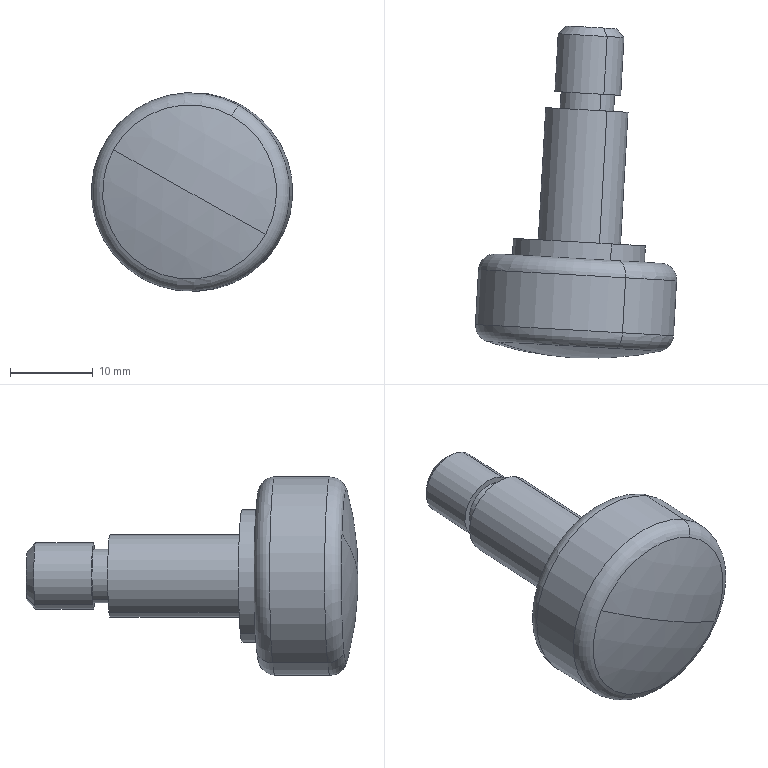Component | SolidWorks | Foot-1 | 1 solid | 23 faces | box 24.34 x 40.17 x 24 mm | volume 7037 mm3 | cylinder 10 | plane 5 | torus 4 | cone 2 | sphere 2 | commonest cylinder face diameters 24 x2 16 x2 10 x2 6.5 x2 8 x2
build123d program:
from build123d import *

# Parameters (mm, degrees)
CHAMFER1_SIZE = 1


with BuildPart() as part:
    # Sketch1 → Revolve1 (revolve)
    with BuildSketch(Plane.XY, mode=Mode.PRIVATE) as revolve1_sk:
        with BuildLine():
            Line((3.339, 12), (10, 12))
            ThreePointArc((10, 12), (11.414, 11.414), (12, 10))
            Line((12, 10), (12, 8))
            Line((12, 8), (14, 8))
            Line((14, 8), (14, 5))
            Line((14, 5), (30, 5))
            Line((30, 5), (30, 3.25))
            Line((30, 3.25), (32, 3.25))
            Line((32, 3.25), (32, 4))
            Line((32, 4), (40, 4))
            Line((40, 4), (40, 0))
            Line((40, 0), (0, 0))
            ThreePointArc((0, 0), (0.354, 5.31), (1.41, 10.526))
            ThreePointArc((1.41, 10.526), (2.125, 11.589), (3.339, 12))
        make_face()
    revolve(revolve1_sk.sketch.rotate(Axis((0, 0, 0), (1, 0, 0)), 90), axis=Axis((0, 0, 0), (1, 0, 0)))

    # Chamfer1
    chamfer1_edges = [part.edges().sort_by_distance(p)[0] for p in [
        (40, 0, -4),
    ]]
    chamfer(chamfer1_edges, length=CHAMFER1_SIZE)


solid = part.part

# Placed as in the assembly
solid = solid.moved(Location((194.855, -53.332, 1009), (-178.207, -28.965, -86.302)))
STEP:
#1=COLOUR_RGB('',0.7922,0.8196,0.9333);
#2=FILL_AREA_STYLE_COLOUR('',#1);
#3=FILL_AREA_STYLE('',(#2));
#4=SURFACE_STYLE_FILL_AREA(#3);
#5=SURFACE_SIDE_STYLE('',(#4));
#6=SURFACE_STYLE_USAGE(.BOTH.,#5);
#7=PRESENTATION_STYLE_ASSIGNMENT((#6));
#8=CARTESIAN_POINT('',(7.703,-0.5241,39.621));
#9=VERTEX_POINT('',#8);
#10=CARTESIAN_POINT('',(7.818,-0.5306,39.828));
#11=VERTEX_POINT('',#10);
#12=CARTESIAN_POINT('',(7.76,-0.5274,39.724));
#13=DIRECTION('',(0.05643,0.9984,0.));
#14=DIRECTION('',(0.4842,-0.02737,0.8745));
#15=AXIS2_PLACEMENT_3D('',#12,#13,#14);
#16=CIRCLE('',#15,0.1181);
#17=EDGE_CURVE('',#9,#11,#16,.T.);
#18=ORIENTED_EDGE('',*,*,#17,.F.);
#19=CARTESIAN_POINT('',(7.682,-0.5624,39.587));
#20=VERTEX_POINT('',#19);
#21=CARTESIAN_POINT('',(7.682,-0.5624,39.587));
#22=DIRECTION('',(-0.3823,-0.6866,-0.6184));
#23=VECTOR('',#22,39.37);
#24=LINE('',#21,#23);
#25=EDGE_CURVE('',#9,#20,#24,.T.);
#26=ORIENTED_EDGE('',*,*,#25,.T.);
#27=CARTESIAN_POINT('',(7.834,-0.571,39.862));
#28=VERTEX_POINT('',#27);
#29=CARTESIAN_POINT('',(7.758,-0.5667,39.724));
#30=DIRECTION('',(-0.05643,-0.9984,-0.));
#31=DIRECTION('',(0.4842,-0.02737,0.8745));
#32=AXIS2_PLACEMENT_3D('',#29,#30,#31);
#33=CIRCLE('',#32,0.1575);
#34=EDGE_CURVE('',#28,#20,#33,.T.);
#35=ORIENTED_EDGE('',*,*,#34,.F.);
#36=CARTESIAN_POINT('',(7.834,-0.571,39.862));
#37=DIRECTION('',(0.3025,-0.7253,0.6184));
#38=VECTOR('',#37,39.37);
#39=LINE('',#36,#38);
#40=EDGE_CURVE('',#11,#28,#39,.T.);
#41=ORIENTED_EDGE('',*,*,#40,.F.);
#42=EDGE_LOOP('',(#18,#26,#35,#41));
#43=FACE_OUTER_BOUND('',#42,.T.);
#44=CARTESIAN_POINT('',(7.758,-0.5667,39.724));
#45=DIRECTION('',(-0.05643,-0.9984,-0.));
#46=DIRECTION('',(0.4842,-0.02737,0.8745));
#47=AXIS2_PLACEMENT_3D('',#44,#45,#46);
#48=CONICAL_SURFACE('',#47,0.1575,0.7854);
#49=ADVANCED_FACE('',(#43),#48,.T.);
#50=CARTESIAN_POINT('',(7.908,-1.981,40.138));
#51=VERTEX_POINT('',#50);
#52=CARTESIAN_POINT('',(7.45,-1.955,39.311));
#53=VERTEX_POINT('',#52);
#54=CARTESIAN_POINT('',(7.679,-1.968,39.724));
#55=DIRECTION('',(-0.05643,-0.9984,-0.));
#56=DIRECTION('',(0.4842,-0.02737,0.8745));
#57=AXIS2_PLACEMENT_3D('',#54,#55,#56);
#58=CIRCLE('',#57,0.4724);
#59=EDGE_CURVE('',#51,#53,#58,.T.);
#60=ORIENTED_EDGE('',*,*,#59,.T.);
#61=CARTESIAN_POINT('',(7.474,-2.033,39.362));
#62=VERTEX_POINT('',#61);
#63=CARTESIAN_POINT('',(7.488,-1.958,39.38));
#64=DIRECTION('',(-0.8731,0.04935,0.485));
#65=DIRECTION('',(0.4856,0.,0.8742));
#66=AXIS2_PLACEMENT_3D('',#63,#64,#65);
#67=CIRCLE('',#66,0.07874);
#68=EDGE_CURVE('',#53,#62,#67,.T.);
#69=ORIENTED_EDGE('',*,*,#68,.T.);
#70=CARTESIAN_POINT('',(7.313,-2.024,39.925));
#71=VERTEX_POINT('',#70);
#72=CARTESIAN_POINT('',(7.675,-2.044,39.724));
#73=DIRECTION('',(-0.05643,-0.9984,-0.));
#74=DIRECTION('',(0.4842,-0.02737,0.8745));
#75=AXIS2_PLACEMENT_3D('',#72,#73,#74);
#76=CIRCLE('',#75,0.4144);
#77=EDGE_CURVE('',#71,#62,#76,.T.);
#78=ORIENTED_EDGE('',*,*,#77,.F.);
#79=CARTESIAN_POINT('',(7.875,-2.056,40.087));
#80=VERTEX_POINT('',#79);
#81=CARTESIAN_POINT('',(7.675,-2.044,39.724));
#82=DIRECTION('',(-0.05643,-0.9984,-0.));
#83=DIRECTION('',(0.4842,-0.02737,0.8745));
#84=AXIS2_PLACEMENT_3D('',#81,#82,#83);
#85=CIRCLE('',#84,0.4144);
#86=EDGE_CURVE('',#80,#71,#85,.T.);
#87=ORIENTED_EDGE('',*,*,#86,.F.);
#88=CARTESIAN_POINT('',(7.87,-1.979,40.069));
#89=DIRECTION('',(0.8731,-0.04935,-0.485));
#90=DIRECTION('',(-0.4856,0.,-0.8742));
#91=AXIS2_PLACEMENT_3D('',#88,#89,#90);
#92=CIRCLE('',#91,0.07874);
#93=EDGE_CURVE('',#51,#80,#92,.T.);
#94=ORIENTED_EDGE('',*,*,#93,.F.);
#95=EDGE_LOOP('',(#60,#69,#78,#87,#94));
#96=FACE_OUTER_BOUND('',#95,.T.);
#97=CARTESIAN_POINT('',(7.679,-1.968,39.724));
#98=DIRECTION('',(-0.05643,-0.9984,-0.));
#99=DIRECTION('',(0.4842,-0.02737,0.8745));
#100=AXIS2_PLACEMENT_3D('',#97,#98,#99);
#101=TOROIDAL_SURFACE('',#100,0.3937,0.07874);
#102=ADVANCED_FACE('',(#96),#101,.T.);
#103=CARTESIAN_POINT('',(7.922,-1.72,40.138));
#104=VERTEX_POINT('',#103);
#105=CARTESIAN_POINT('',(7.465,-1.694,39.311));
#106=VERTEX_POINT('',#105);
#107=CARTESIAN_POINT('',(7.694,-1.707,39.724));
#108=DIRECTION('',(-0.05643,-0.9984,-0.));
#109=DIRECTION('',(0.4842,-0.02737,0.8745));
#110=AXIS2_PLACEMENT_3D('',#107,#108,#109);
#111=CIRCLE('',#110,0.4724);
#112=EDGE_CURVE('',#104,#106,#111,.T.);
#113=ORIENTED_EDGE('',*,*,#112,.T.);
#114=CARTESIAN_POINT('',(7.443,-2.087,39.311));
#115=DIRECTION('',(-0.05643,-0.9984,-0.));
#116=VECTOR('',#115,39.37);
#117=LINE('',#114,#116);
#118=EDGE_CURVE('',#106,#53,#117,.T.);
#119=ORIENTED_EDGE('',*,*,#118,.T.);
#120=ORIENTED_EDGE('',*,*,#59,.F.);
#121=CARTESIAN_POINT('',(7.9,-2.113,40.138));
#122=DIRECTION('',(-0.05643,-0.9984,-0.));
#123=VECTOR('',#122,39.37);
#124=LINE('',#121,#123);
#125=EDGE_CURVE('',#104,#51,#124,.T.);
#126=ORIENTED_EDGE('',*,*,#125,.F.);
#127=EDGE_LOOP('',(#113,#119,#120,#126));
#128=FACE_OUTER_BOUND('',#127,.T.);
#129=CARTESIAN_POINT('',(7.671,-2.1,39.724));
#130=DIRECTION('',(-0.05643,-0.9984,-0.));
#131=DIRECTION('',(0.4842,-0.02737,0.8745));
#132=AXIS2_PLACEMENT_3D('',#129,#130,#131);
#133=CYLINDRICAL_SURFACE('',#132,0.4724);
#134=ADVANCED_FACE('',(#128),#133,.T.);
#135=CARTESIAN_POINT('',(7.889,-1.639,40.069));
#136=VERTEX_POINT('',#135);
#137=CARTESIAN_POINT('',(7.508,-1.617,39.38));
#138=VERTEX_POINT('',#137);
#139=CARTESIAN_POINT('',(7.698,-1.628,39.724));
#140=DIRECTION('',(-0.05643,-0.9984,-0.));
#141=DIRECTION('',(0.4842,-0.02737,0.8745));
#142=AXIS2_PLACEMENT_3D('',#139,#140,#141);
#143=CIRCLE('',#142,0.3937);
#144=EDGE_CURVE('',#136,#138,#143,.T.);
#145=ORIENTED_EDGE('',*,*,#144,.T.);
#146=CARTESIAN_POINT('',(7.503,-1.696,39.38));
#147=DIRECTION('',(-0.8731,0.04935,0.485));
#148=DIRECTION('',(0.4856,0.,0.8742));
#149=AXIS2_PLACEMENT_3D('',#146,#147,#148);
#150=CIRCLE('',#149,0.07874);
#151=EDGE_CURVE('',#138,#106,#150,.T.);
#152=ORIENTED_EDGE('',*,*,#151,.T.);
#153=ORIENTED_EDGE('',*,*,#112,.F.);
#154=CARTESIAN_POINT('',(7.884,-1.717,40.069));
#155=DIRECTION('',(0.8731,-0.04935,-0.485));
#156=DIRECTION('',(-0.4856,0.,-0.8742));
#157=AXIS2_PLACEMENT_3D('',#154,#155,#156);
#158=CIRCLE('',#157,0.07874);
#159=EDGE_CURVE('',#136,#104,#158,.T.);
#160=ORIENTED_EDGE('',*,*,#159,.F.);
#161=EDGE_LOOP('',(#145,#152,#153,#160));
#162=FACE_OUTER_BOUND('',#161,.T.);
#163=CARTESIAN_POINT('',(7.694,-1.707,39.724));
#164=DIRECTION('',(-0.05643,-0.9984,-0.));
#165=DIRECTION('',(0.4842,-0.02737,0.8745));
#166=AXIS2_PLACEMENT_3D('',#163,#164,#165);
#167=TOROIDAL_SURFACE('',#166,0.3937,0.07874);
#168=ADVANCED_FACE('',(#162),#167,.T.);
#169=CARTESIAN_POINT('',(7.855,-1.558,40.));
#170=VERTEX_POINT('',#169);
#171=CARTESIAN_POINT('',(7.55,-1.541,39.449));
#172=VERTEX_POINT('',#171);
#173=CARTESIAN_POINT('',(7.703,-1.549,39.724));
#174=DIRECTION('',(-0.05643,-0.9984,-0.));
#175=DIRECTION('',(0.4842,-0.02737,0.8745));
#176=AXIS2_PLACEMENT_3D('',#173,#174,#175);
#177=CIRCLE('',#176,0.315);
#178=EDGE_CURVE('',#170,#172,#177,.T.);
#179=ORIENTED_EDGE('',*,*,#178,.T.);
#180=CARTESIAN_POINT('',(7.546,-1.619,39.449));
#181=VERTEX_POINT('',#180);
#182=CARTESIAN_POINT('',(7.519,-2.091,39.449));
#183=DIRECTION('',(-0.05643,-0.9984,-0.));
#184=VECTOR('',#183,39.37);
#185=LINE('',#182,#184);
#186=EDGE_CURVE('',#172,#181,#185,.T.);
#187=ORIENTED_EDGE('',*,*,#186,.T.);
#188=CARTESIAN_POINT('',(7.851,-1.637,40.));
#189=VERTEX_POINT('',#188);
#190=CARTESIAN_POINT('',(7.698,-1.628,39.724));
#191=DIRECTION('',(-0.05643,-0.9984,-0.));
#192=DIRECTION('',(0.4842,-0.02737,0.8745));
#193=AXIS2_PLACEMENT_3D('',#190,#191,#192);
#194=CIRCLE('',#193,0.315);
#195=EDGE_CURVE('',#189,#181,#194,.T.);
#196=ORIENTED_EDGE('',*,*,#195,.F.);
#197=CARTESIAN_POINT('',(7.824,-2.108,40.));
#198=DIRECTION('',(-0.05643,-0.9984,-0.));
#199=VECTOR('',#198,39.37);
#200=LINE('',#197,#199);
#201=EDGE_CURVE('',#170,#189,#200,.T.);
#202=ORIENTED_EDGE('',*,*,#201,.F.);
#203=EDGE_LOOP('',(#179,#187,#196,#202));
#204=FACE_OUTER_BOUND('',#203,.T.);
#205=CARTESIAN_POINT('',(7.671,-2.1,39.724));
#206=DIRECTION('',(-0.05643,-0.9984,-0.));
#207=DIRECTION('',(0.4842,-0.02737,0.8745));
#208=AXIS2_PLACEMENT_3D('',#205,#206,#207);
#209=CYLINDRICAL_SURFACE('',#208,0.315);
#210=ADVANCED_FACE('',(#204),#209,.T.);
#211=CARTESIAN_POINT('',(7.833,-0.9258,39.897));
#212=VERTEX_POINT('',#211);
#213=CARTESIAN_POINT('',(7.643,-0.9151,39.552));
#214=VERTEX_POINT('',#213);
#215=CARTESIAN_POINT('',(7.738,-0.9205,39.724));
#216=DIRECTION('',(-0.05643,-0.9984,-0.));
#217=DIRECTION('',(0.4842,-0.02737,0.8745));
#218=AXIS2_PLACEMENT_3D('',#215,#216,#217);
#219=CIRCLE('',#218,0.1969);
#220=EDGE_CURVE('',#212,#214,#219,.T.);
#221=ORIENTED_EDGE('',*,*,#220,.T.);
#222=CARTESIAN_POINT('',(7.607,-1.544,39.552));
#223=VERTEX_POINT('',#222);
#224=CARTESIAN_POINT('',(7.576,-2.094,39.552));
#225=DIRECTION('',(-0.05643,-0.9984,-0.));
#226=VECTOR('',#225,39.37);
#227=LINE('',#224,#226);
#228=EDGE_CURVE('',#214,#223,#227,.T.);
#229=ORIENTED_EDGE('',*,*,#228,.T.);
#230=CARTESIAN_POINT('',(7.798,-1.555,39.897));
#231=VERTEX_POINT('',#230);
#232=CARTESIAN_POINT('',(7.703,-1.549,39.724));
#233=DIRECTION('',(-0.05643,-0.9984,-0.));
#234=DIRECTION('',(0.4842,-0.02737,0.8745));
#235=AXIS2_PLACEMENT_3D('',#232,#233,#234);
#236=CIRCLE('',#235,0.1969);
#237=EDGE_CURVE('',#231,#223,#236,.T.);
#238=ORIENTED_EDGE('',*,*,#237,.F.);
#239=CARTESIAN_POINT('',(7.767,-2.105,39.897));
#240=DIRECTION('',(-0.05643,-0.9984,-0.));
#241=VECTOR('',#240,39.37);
#242=LINE('',#239,#241);
#243=EDGE_CURVE('',#212,#231,#242,.T.);
#244=ORIENTED_EDGE('',*,*,#243,.F.);
#245=EDGE_LOOP('',(#221,#229,#238,#244));
#246=FACE_OUTER_BOUND('',#245,.T.);
#247=CARTESIAN_POINT('',(7.671,-2.1,39.724));
#248=DIRECTION('',(-0.05643,-0.9984,-0.));
#249=DIRECTION('',(0.4842,-0.02737,0.8745));
#250=AXIS2_PLACEMENT_3D('',#247,#248,#249);
#251=CYLINDRICAL_SURFACE('',#250,0.1969);
#252=ADVANCED_FACE('',(#246),#251,.T.);
#253=CARTESIAN_POINT('',(7.805,-0.8453,39.836));
#254=VERTEX_POINT('',#253);
#255=CARTESIAN_POINT('',(7.681,-0.8383,39.613));
#256=VERTEX_POINT('',#255);
#257=CARTESIAN_POINT('',(7.743,-0.8418,39.724));
#258=DIRECTION('',(-0.05643,-0.9984,-0.));
#259=DIRECTION('',(0.4842,-0.02737,0.8745));
#260=AXIS2_PLACEMENT_3D('',#257,#258,#259);
#261=CIRCLE('',#260,0.128);
#262=EDGE_CURVE('',#254,#256,#261,.T.);
#263=ORIENTED_EDGE('',*,*,#262,.T.);
#264=CARTESIAN_POINT('',(7.676,-0.9169,39.613));
#265=VERTEX_POINT('',#264);
#266=CARTESIAN_POINT('',(7.61,-2.096,39.613));
#267=DIRECTION('',(-0.05643,-0.9984,-0.));
#268=VECTOR('',#267,39.37);
#269=LINE('',#266,#268);
#270=EDGE_CURVE('',#256,#265,#269,.T.);
#271=ORIENTED_EDGE('',*,*,#270,.T.);
#272=CARTESIAN_POINT('',(7.8,-0.924,39.836));
#273=VERTEX_POINT('',#272);
#274=CARTESIAN_POINT('',(7.738,-0.9205,39.724));
#275=DIRECTION('',(-0.05643,-0.9984,-0.));
#276=DIRECTION('',(0.4842,-0.02737,0.8745));
#277=AXIS2_PLACEMENT_3D('',#274,#275,#276);
#278=CIRCLE('',#277,0.128);
#279=EDGE_CURVE('',#273,#265,#278,.T.);
#280=ORIENTED_EDGE('',*,*,#279,.F.);
#281=CARTESIAN_POINT('',(7.733,-2.103,39.836));
#282=DIRECTION('',(-0.05643,-0.9984,-0.));
#283=VECTOR('',#282,39.37);
#284=LINE('',#281,#283);
#285=EDGE_CURVE('',#254,#273,#284,.T.);
#286=ORIENTED_EDGE('',*,*,#285,.F.);
#287=EDGE_LOOP('',(#263,#271,#280,#286));
#288=FACE_OUTER_BOUND('',#287,.T.);
#289=CARTESIAN_POINT('',(7.671,-2.1,39.724));
#290=DIRECTION('',(-0.05643,-0.9984,-0.));
#291=DIRECTION('',(0.4842,-0.02737,0.8745));
#292=AXIS2_PLACEMENT_3D('',#289,#290,#291);
#293=CYLINDRICAL_SURFACE('',#292,0.128);
#294=ADVANCED_FACE('',(#288),#293,.T.);
#295=ORIENTED_EDGE('',*,*,#34,.T.);
#296=CARTESIAN_POINT('',(7.666,-0.8375,39.587));
#297=VERTEX_POINT('',#296);
#298=CARTESIAN_POINT('',(7.595,-2.095,39.587));
#299=DIRECTION('',(-0.05643,-0.9984,-0.));
#300=VECTOR('',#299,39.37);
#301=LINE('',#298,#300);
#302=EDGE_CURVE('',#20,#297,#301,.T.);
#303=ORIENTED_EDGE('',*,*,#302,.T.);
#304=CARTESIAN_POINT('',(7.819,-0.8461,39.862));
#305=VERTEX_POINT('',#304);
#306=CARTESIAN_POINT('',(7.743,-0.8418,39.724));
#307=DIRECTION('',(-0.05643,-0.9984,-0.));
#308=DIRECTION('',(0.4842,-0.02737,0.8745));
#309=AXIS2_PLACEMENT_3D('',#306,#307,#308);
#310=CIRCLE('',#309,0.1575);
#311=EDGE_CURVE('',#305,#297,#310,.T.);
#312=ORIENTED_EDGE('',*,*,#311,.F.);
#313=CARTESIAN_POINT('',(7.748,-2.104,39.862));
#314=DIRECTION('',(-0.05643,-0.9984,-0.));
#315=VECTOR('',#314,39.37);
#316=LINE('',#313,#315);
#317=EDGE_CURVE('',#28,#305,#316,.T.);
#318=ORIENTED_EDGE('',*,*,#317,.F.);
#319=EDGE_LOOP('',(#295,#303,#312,#318));
#320=FACE_OUTER_BOUND('',#319,.T.);
#321=CARTESIAN_POINT('',(7.671,-2.1,39.724));
#322=DIRECTION('',(-0.05643,-0.9984,-0.));
#323=DIRECTION('',(0.4842,-0.02737,0.8745));
#324=AXIS2_PLACEMENT_3D('',#321,#322,#323);
#325=CYLINDRICAL_SURFACE('',#324,0.1575);
#326=ADVANCED_FACE('',(#320),#325,.T.);
#327=ORIENTED_EDGE('',*,*,#77,.T.);
#328=CARTESIAN_POINT('',(8.036,-2.065,39.523));
#329=VERTEX_POINT('',#328);
#330=CARTESIAN_POINT('',(7.675,-2.044,39.724));
#331=DIRECTION('',(-0.05643,-0.9984,-0.));
#332=DIRECTION('',(0.4842,-0.02737,0.8745));
#333=AXIS2_PLACEMENT_3D('',#330,#331,#332);
#334=CIRCLE('',#333,0.4144);
#335=EDGE_CURVE('',#62,#329,#334,.T.);
#336=ORIENTED_EDGE('',*,*,#335,.T.);
#337=CARTESIAN_POINT('',(7.671,-2.1,39.724));
#338=VERTEX_POINT('',#337);
#339=CARTESIAN_POINT('',(7.76,-0.5274,39.724));
#340=DIRECTION('',(-0.4842,0.02737,-0.8745));
#341=DIRECTION('',(-0.8749,0.,0.4844));
#342=AXIS2_PLACEMENT_3D('',#339,#340,#341);
#343=CIRCLE('',#342,1.575);
#344=EDGE_CURVE('',#329,#338,#343,.T.);
#345=ORIENTED_EDGE('',*,*,#344,.T.);
#346=CARTESIAN_POINT('',(7.76,-0.5274,39.724));
#347=DIRECTION('',(0.4842,-0.02737,0.8745));
#348=DIRECTION('',(0.8749,0.,-0.4844));
#349=AXIS2_PLACEMENT_3D('',#346,#347,#348);
#350=CIRCLE('',#349,1.575);
#351=EDGE_CURVE('',#71,#338,#350,.T.);
#352=ORIENTED_EDGE('',*,*,#351,.F.);
#353=EDGE_LOOP('',(#327,#336,#345,#352));
#354=FACE_OUTER_BOUND('',#353,.T.);
#355=CARTESIAN_POINT('',(7.76,-0.5274,39.724));
#356=DIRECTION('',(-0.4842,0.02737,-0.8745));
#357=DIRECTION('',(-0.8731,0.04935,0.485));
#358=AXIS2_PLACEMENT_3D('',#355,#356,#357);
#359=SPHERICAL_SURFACE('',#358,1.575);
#360=ADVANCED_FACE('',(#354),#359,.T.);
#361=ORIENTED_EDGE('',*,*,#344,.F.);
#362=CARTESIAN_POINT('',(7.675,-2.044,39.724));
#363=DIRECTION('',(-0.05643,-0.9984,-0.));
#364=DIRECTION('',(0.4842,-0.02737,0.8745));
#365=AXIS2_PLACEMENT_3D('',#362,#363,#364);
#366=CIRCLE('',#365,0.4144);
#367=EDGE_CURVE('',#329,#80,#366,.T.);
#368=ORIENTED_EDGE('',*,*,#367,.T.);
#369=ORIENTED_EDGE('',*,*,#86,.T.);
#370=ORIENTED_EDGE('',*,*,#351,.T.);
#371=EDGE_LOOP('',(#361,#368,#369,#370));
#372=FACE_OUTER_BOUND('',#371,.T.);
#373=CARTESIAN_POINT('',(7.76,-0.5274,39.724));
#374=DIRECTION('',(-0.4842,0.02737,-0.8745));
#375=DIRECTION('',(-0.8731,0.04935,0.485));
#376=AXIS2_PLACEMENT_3D('',#373,#374,#375);
#377=SPHERICAL_SURFACE('',#376,1.575);
#378=ADVANCED_FACE('',(#372),#377,.T.);
#379=CARTESIAN_POINT('',(7.76,-0.5274,39.724));
#380=DIRECTION('',(0.05643,0.9984,0.));
#381=DIRECTION('',(0.4842,-0.02737,0.8745));
#382=AXIS2_PLACEMENT_3D('',#379,#380,#381);
#383=CIRCLE('',#382,0.1181);
#384=EDGE_CURVE('',#11,#9,#383,.T.);
#385=ORIENTED_EDGE('',*,*,#384,.T.);
#386=ORIENTED_EDGE('',*,*,#17,.T.);
#387=EDGE_LOOP('',(#385,#386));
#388=FACE_OUTER_BOUND('',#387,.T.);
#389=CARTESIAN_POINT('',(7.623,-0.5196,39.801));
#390=DIRECTION('',(-0.05643,-0.9984,-0.));
#391=DIRECTION('',(0.4842,-0.02737,0.8745));
#392=AXIS2_PLACEMENT_3D('',#389,#390,#391);
#393=PLANE('',#392);
#394=ADVANCED_FACE('',(#388),#393,.F.);
#395=ORIENTED_EDGE('',*,*,#302,.F.);
#396=CARTESIAN_POINT('',(7.758,-0.5667,39.724));
#397=DIRECTION('',(-0.05643,-0.9984,-0.));
#398=DIRECTION('',(0.4842,-0.02737,0.8745));
#399=AXIS2_PLACEMENT_3D('',#396,#397,#398);
#400=CIRCLE('',#399,0.1575);
#401=EDGE_CURVE('',#20,#28,#400,.T.);
#402=ORIENTED_EDGE('',*,*,#401,.T.);
#403=ORIENTED_EDGE('',*,*,#317,.T.);
#404=CARTESIAN_POINT('',(7.743,-0.8418,39.724));
#405=DIRECTION('',(-0.05643,-0.9984,-0.));
#406=DIRECTION('',(0.4842,-0.02737,0.8745));
#407=AXIS2_PLACEMENT_3D('',#404,#405,#406);
#408=CIRCLE('',#407,0.1575);
#409=EDGE_CURVE('',#297,#305,#408,.T.);
#410=ORIENTED_EDGE('',*,*,#409,.F.);
#411=EDGE_LOOP('',(#395,#402,#403,#410));
#412=FACE_OUTER_BOUND('',#411,.T.);
#413=CARTESIAN_POINT('',(7.671,-2.1,39.724));
#414=DIRECTION('',(-0.05643,-0.9984,-0.));
#415=DIRECTION('',(0.4842,-0.02737,0.8745));
#416=AXIS2_PLACEMENT_3D('',#413,#414,#415);
#417=CYLINDRICAL_SURFACE('',#416,0.1575);
#418=ADVANCED_FACE('',(#412),#417,.T.);
#419=ORIENTED_EDGE('',*,*,#262,.F.);
#420=CARTESIAN_POINT('',(7.743,-0.8418,39.724));
#421=DIRECTION('',(-0.05643,-0.9984,-0.));
#422=DIRECTION('',(0.4842,-0.02737,0.8745));
#423=AXIS2_PLACEMENT_3D('',#420,#421,#422);
#424=CIRCLE('',#423,0.128);
#425=EDGE_CURVE('',#256,#254,#424,.T.);
#426=ORIENTED_EDGE('',*,*,#425,.F.);
#427=EDGE_LOOP('',(#419,#426));
#428=FACE_BOUND('',#427,.T.);
#429=ORIENTED_EDGE('',*,*,#311,.T.);
#430=ORIENTED_EDGE('',*,*,#409,.T.);
#431=EDGE_LOOP('',(#429,#430));
#432=FACE_OUTER_BOUND('',#431,.T.);
#433=CARTESIAN_POINT('',(7.631,-0.8355,39.786));
#434=DIRECTION('',(0.05643,0.9984,0.));
#435=DIRECTION('',(-0.4842,0.02737,-0.8745));
#436=AXIS2_PLACEMENT_3D('',#433,#434,#435);
#437=PLANE('',#436);
#438=ADVANCED_FACE('',(#428,#432),#437,.F.);
#439=ORIENTED_EDGE('',*,*,#270,.F.);
#440=ORIENTED_EDGE('',*,*,#425,.T.);
#441=ORIENTED_EDGE('',*,*,#285,.T.);
#442=CARTESIAN_POINT('',(7.738,-0.9205,39.724));
#443=DIRECTION('',(-0.05643,-0.9984,-0.));
#444=DIRECTION('',(0.4842,-0.02737,0.8745));
#445=AXIS2_PLACEMENT_3D('',#442,#443,#444);
#446=CIRCLE('',#445,0.128);
#447=EDGE_CURVE('',#265,#273,#446,.T.);
#448=ORIENTED_EDGE('',*,*,#447,.F.);
#449=EDGE_LOOP('',(#439,#440,#441,#448));
#450=FACE_OUTER_BOUND('',#449,.T.);
#451=CARTESIAN_POINT('',(7.671,-2.1,39.724));
#452=DIRECTION('',(-0.05643,-0.9984,-0.));
#453=DIRECTION('',(0.4842,-0.02737,0.8745));
#454=AXIS2_PLACEMENT_3D('',#451,#452,#453);
#455=CYLINDRICAL_SURFACE('',#454,0.128);
#456=ADVANCED_FACE('',(#450),#455,.T.);
#457=ORIENTED_EDGE('',*,*,#220,.F.);
#458=CARTESIAN_POINT('',(7.738,-0.9205,39.724));
#459=DIRECTION('',(-0.05643,-0.9984,-0.));
#460=DIRECTION('',(0.4842,-0.02737,0.8745));
#461=AXIS2_PLACEMENT_3D('',#458,#459,#460);
#462=CIRCLE('',#461,0.1969);
#463=EDGE_CURVE('',#214,#212,#462,.T.);
#464=ORIENTED_EDGE('',*,*,#463,.F.);
#465=EDGE_LOOP('',(#457,#464));
#466=FACE_OUTER_BOUND('',#465,.T.);
#467=ORIENTED_EDGE('',*,*,#279,.T.);
#468=ORIENTED_EDGE('',*,*,#447,.T.);
#469=EDGE_LOOP('',(#467,#468));
#470=FACE_BOUND('',#469,.T.);
#471=CARTESIAN_POINT('',(7.566,-0.9107,39.82));
#472=DIRECTION('',(-0.05643,-0.9984,-0.));
#473=DIRECTION('',(0.4842,-0.02737,0.8745));
#474=AXIS2_PLACEMENT_3D('',#471,#472,#473);
#475=PLANE('',#474);
#476=ADVANCED_FACE('',(#466,#470),#475,.F.);
#477=ORIENTED_EDGE('',*,*,#228,.F.);
#478=ORIENTED_EDGE('',*,*,#463,.T.);
#479=ORIENTED_EDGE('',*,*,#243,.T.);
#480=CARTESIAN_POINT('',(7.703,-1.549,39.724));
#481=DIRECTION('',(-0.05643,-0.9984,-0.));
#482=DIRECTION('',(0.4842,-0.02737,0.8745));
#483=AXIS2_PLACEMENT_3D('',#480,#481,#482);
#484=CIRCLE('',#483,0.1969);
#485=EDGE_CURVE('',#223,#231,#484,.T.);
#486=ORIENTED_EDGE('',*,*,#485,.F.);
#487=EDGE_LOOP('',(#477,#478,#479,#486));
#488=FACE_OUTER_BOUND('',#487,.T.);
#489=CARTESIAN_POINT('',(7.671,-2.1,39.724));
#490=DIRECTION('',(-0.05643,-0.9984,-0.));
#491=DIRECTION('',(0.4842,-0.02737,0.8745));
#492=AXIS2_PLACEMENT_3D('',#489,#490,#491);
#493=CYLINDRICAL_SURFACE('',#492,0.1969);
#494=ADVANCED_FACE('',(#488),#493,.T.);
#495=ORIENTED_EDGE('',*,*,#178,.F.);
#496=CARTESIAN_POINT('',(7.703,-1.549,39.724));
#497=DIRECTION('',(-0.05643,-0.9984,-0.));
#498=DIRECTION('',(0.4842,-0.02737,0.8745));
#499=AXIS2_PLACEMENT_3D('',#496,#497,#498);
#500=CIRCLE('',#499,0.315);
#501=EDGE_CURVE('',#172,#170,#500,.T.);
#502=ORIENTED_EDGE('',*,*,#501,.F.);
#503=EDGE_LOOP('',(#495,#502));
#504=FACE_OUTER_BOUND('',#503,.T.);
#505=ORIENTED_EDGE('',*,*,#237,.T.);
#506=ORIENTED_EDGE('',*,*,#485,.T.);
#507=EDGE_LOOP('',(#505,#506));
#508=FACE_BOUND('',#507,.T.);
#509=CARTESIAN_POINT('',(7.428,-1.534,39.877));
#510=DIRECTION('',(-0.05643,-0.9984,-0.));
#511=DIRECTION('',(0.4842,-0.02737,0.8745));
#512=AXIS2_PLACEMENT_3D('',#509,#510,#511);
#513=PLANE('',#512);
#514=ADVANCED_FACE('',(#504,#508),#513,.F.);
#515=ORIENTED_EDGE('',*,*,#186,.F.);
#516=ORIENTED_EDGE('',*,*,#501,.T.);
#517=ORIENTED_EDGE('',*,*,#201,.T.);
#518=CARTESIAN_POINT('',(7.698,-1.628,39.724));
#519=DIRECTION('',(-0.05643,-0.9984,-0.));
#520=DIRECTION('',(0.4842,-0.02737,0.8745));
#521=AXIS2_PLACEMENT_3D('',#518,#519,#520);
#522=CIRCLE('',#521,0.315);
#523=EDGE_CURVE('',#181,#189,#522,.T.);
#524=ORIENTED_EDGE('',*,*,#523,.F.);
#525=EDGE_LOOP('',(#515,#516,#517,#524));
#526=FACE_OUTER_BOUND('',#525,.T.);
#527=CARTESIAN_POINT('',(7.671,-2.1,39.724));
#528=DIRECTION('',(-0.05643,-0.9984,-0.));
#529=DIRECTION('',(0.4842,-0.02737,0.8745));
#530=AXIS2_PLACEMENT_3D('',#527,#528,#529);
#531=CYLINDRICAL_SURFACE('',#530,0.315);
#532=ADVANCED_FACE('',(#526),#531,.T.);
#533=ORIENTED_EDGE('',*,*,#144,.F.);
#534=CARTESIAN_POINT('',(7.698,-1.628,39.724));
#535=DIRECTION('',(-0.05643,-0.9984,-0.));
#536=DIRECTION('',(0.4842,-0.02737,0.8745));
#537=AXIS2_PLACEMENT_3D('',#534,#535,#536);
#538=CIRCLE('',#537,0.3937);
#539=EDGE_CURVE('',#138,#136,#538,.T.);
#540=ORIENTED_EDGE('',*,*,#539,.F.);
#541=EDGE_LOOP('',(#533,#540));
#542=FACE_OUTER_BOUND('',#541,.T.);
#543=ORIENTED_EDGE('',*,*,#195,.T.);
#544=ORIENTED_EDGE('',*,*,#523,.T.);
#545=EDGE_LOOP('',(#543,#544));
#546=FACE_BOUND('',#545,.T.);
#547=CARTESIAN_POINT('',(7.354,-1.609,39.915));
#548=DIRECTION('',(-0.05643,-0.9984,-0.));
#549=DIRECTION('',(0.4842,-0.02737,0.8745));
#550=AXIS2_PLACEMENT_3D('',#547,#548,#549);
#551=PLANE('',#550);
#552=ADVANCED_FACE('',(#542,#546),#551,.F.);
#553=ORIENTED_EDGE('',*,*,#151,.F.);
#554=ORIENTED_EDGE('',*,*,#539,.T.);
#555=ORIENTED_EDGE('',*,*,#159,.T.);
#556=CARTESIAN_POINT('',(7.694,-1.707,39.724));
#557=DIRECTION('',(-0.05643,-0.9984,-0.));
#558=DIRECTION('',(0.4842,-0.02737,0.8745));
#559=AXIS2_PLACEMENT_3D('',#556,#557,#558);
#560=CIRCLE('',#559,0.4724);
#561=EDGE_CURVE('',#106,#104,#560,.T.);
#562=ORIENTED_EDGE('',*,*,#561,.F.);
#563=EDGE_LOOP('',(#553,#554,#555,#562));
#564=FACE_OUTER_BOUND('',#563,.T.);
#565=CARTESIAN_POINT('',(7.694,-1.707,39.724));
#566=DIRECTION('',(-0.05643,-0.9984,-0.));
#567=DIRECTION('',(0.4842,-0.02737,0.8745));
#568=AXIS2_PLACEMENT_3D('',#565,#566,#567);
#569=TOROIDAL_SURFACE('',#568,0.3937,0.07874);
#570=ADVANCED_FACE('',(#564),#569,.T.);
#571=ORIENTED_EDGE('',*,*,#118,.F.);
#572=ORIENTED_EDGE('',*,*,#561,.T.);
#573=ORIENTED_EDGE('',*,*,#125,.T.);
#574=CARTESIAN_POINT('',(7.679,-1.968,39.724));
#575=DIRECTION('',(-0.05643,-0.9984,-0.));
#576=DIRECTION('',(0.4842,-0.02737,0.8745));
#577=AXIS2_PLACEMENT_3D('',#574,#575,#576);
#578=CIRCLE('',#577,0.4724);
#579=EDGE_CURVE('',#53,#51,#578,.T.);
#580=ORIENTED_EDGE('',*,*,#579,.F.);
#581=EDGE_LOOP('',(#571,#572,#573,#580));
#582=FACE_OUTER_BOUND('',#581,.T.);
#583=CARTESIAN_POINT('',(7.671,-2.1,39.724));
#584=DIRECTION('',(-0.05643,-0.9984,-0.));
#585=DIRECTION('',(0.4842,-0.02737,0.8745));
#586=AXIS2_PLACEMENT_3D('',#583,#584,#585);
#587=CYLINDRICAL_SURFACE('',#586,0.4724);
#588=ADVANCED_FACE('',(#582),#587,.T.);
#589=ORIENTED_EDGE('',*,*,#68,.F.);
#590=ORIENTED_EDGE('',*,*,#579,.T.);
#591=ORIENTED_EDGE('',*,*,#93,.T.);
#592=ORIENTED_EDGE('',*,*,#367,.F.);
#593=ORIENTED_EDGE('',*,*,#335,.F.);
#594=EDGE_LOOP('',(#589,#590,#591,#592,#593));
#595=FACE_OUTER_BOUND('',#594,.T.);
#596=CARTESIAN_POINT('',(7.679,-1.968,39.724));
#597=DIRECTION('',(-0.05643,-0.9984,-0.));
#598=DIRECTION('',(0.4842,-0.02737,0.8745));
#599=AXIS2_PLACEMENT_3D('',#596,#597,#598);
#600=TOROIDAL_SURFACE('',#599,0.3937,0.07874);
#601=ADVANCED_FACE('',(#595),#600,.T.);
#602=ORIENTED_EDGE('',*,*,#25,.F.);
#603=ORIENTED_EDGE('',*,*,#384,.F.);
#604=ORIENTED_EDGE('',*,*,#40,.T.);
#605=ORIENTED_EDGE('',*,*,#401,.F.);
#606=EDGE_LOOP('',(#602,#603,#604,#605));
#607=FACE_OUTER_BOUND('',#606,.T.);
#608=CARTESIAN_POINT('',(7.758,-0.5667,39.724));
#609=DIRECTION('',(-0.05643,-0.9984,-0.));
#610=DIRECTION('',(0.4842,-0.02737,0.8745));
#611=AXIS2_PLACEMENT_3D('',#608,#609,#610);
#612=CONICAL_SURFACE('',#611,0.1575,0.7854);
#613=ADVANCED_FACE('',(#607),#612,.T.);
#614=CLOSED_SHELL('',(#49,#102,#134,#168,#210,#252,#294,#326,#360,#378,#394,#418,#438,#456,#476,#494,#514,#532,#552,#570,#588,#601,#613));
#615=MANIFOLD_SOLID_BREP('',#614);
#616=STYLED_ITEM('',(#7),#615);
#617=PRESENTATION_LAYER_ASSIGNMENT('','',(#616));
#618=CARTESIAN_POINT('',(0.,0.,0.));
#619=DIRECTION('',(0.,0.,1.));
#620=DIRECTION('',(1.,0.,0.));
#621=AXIS2_PLACEMENT_3D('',#618,#619,#620);
#622=(LENGTH_UNIT()NAMED_UNIT(*)SI_UNIT($,.METRE.));
#623=LENGTH_MEASURE_WITH_UNIT(LENGTH_MEASURE(0.0254),#622);
#624=DIMENSIONAL_EXPONENTS(1.,0.,0.,0.,0.,0.,0.);
#625=(CONVERSION_BASED_UNIT('',#623)LENGTH_UNIT()NAMED_UNIT(#624));
#626=UNCERTAINTY_MEASURE_WITH_UNIT(LENGTH_MEASURE(0.00001),#625,'','');
#627=(NAMED_UNIT(*)PLANE_ANGLE_UNIT()SI_UNIT($,.RADIAN.));
#628=(NAMED_UNIT(*)SI_UNIT($,.STERADIAN.)SOLID_ANGLE_UNIT());
#629=(GEOMETRIC_REPRESENTATION_CONTEXT(3)GLOBAL_UNCERTAINTY_ASSIGNED_CONTEXT((#626))GLOBAL_UNIT_ASSIGNED_CONTEXT((#625,#627,#628))REPRESENTATION_CONTEXT('',''));
#630=ADVANCED_BREP_SHAPE_REPRESENTATION('',(#615,#621),#629);
#631=(LENGTH_UNIT()NAMED_UNIT(*)SI_UNIT($,.METRE.));
#632=LENGTH_MEASURE_WITH_UNIT(LENGTH_MEASURE(0.0254),#631);
#633=DIMENSIONAL_EXPONENTS(1.,0.,0.,0.,0.,0.,0.);
#634=(CONVERSION_BASED_UNIT('',#632)LENGTH_UNIT()NAMED_UNIT(#633));
#635=UNCERTAINTY_MEASURE_WITH_UNIT(LENGTH_MEASURE(0.00001),#634,'','');
#636=(NAMED_UNIT(*)PLANE_ANGLE_UNIT()SI_UNIT($,.RADIAN.));
#637=(NAMED_UNIT(*)SI_UNIT($,.STERADIAN.)SOLID_ANGLE_UNIT());
#638=(GEOMETRIC_REPRESENTATION_CONTEXT(3)GLOBAL_UNCERTAINTY_ASSIGNED_CONTEXT((#635))GLOBAL_UNIT_ASSIGNED_CONTEXT((#634,#636,#637))REPRESENTATION_CONTEXT('',''));
#639=MECHANICAL_DESIGN_GEOMETRIC_PRESENTATION_REPRESENTATION('',(#616),#638);